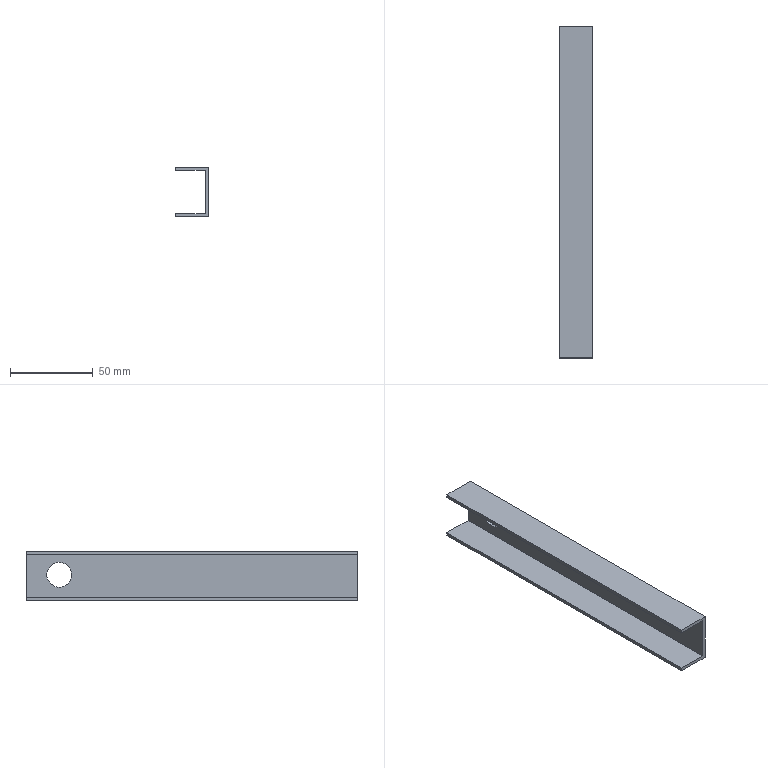Component | SolidWorks | Copy_of_Part4-1 | 1 solid | 12 faces | box 20 x 200 x 30 mm | volume 26047 mm3 | plane 10 | cylinder 2 | commonest cylinder face diameters 15 x2
build123d program:
from build123d import *

# Parameters (mm, degrees)
EXTRUDE_THIN1_DEPTH = 200
SKETCH3_R           = 7.5
CUT_EXTRUDE1_DEPTH  = 254


with BuildPart() as part:
    # Sketch2 → Extrude-Thin1 (new body)
    with BuildSketch(Plane(origin=(0, 0, 0), x_dir=(1, 0, 0), z_dir=(0, 1, 0))):
        Polygon((-173.819, 20), (-173.819, 0), (-143.819, 0), (-143.819, 20), (-145.819, 20), (-145.819, 2), (-171.819, 2), (-171.819, 20), align=None)
    extrude(amount=EXTRUDE_THIN1_DEPTH)

    # Sketch3 → Cut-Extrude1 (cut)
    with BuildSketch(Plane.XY):
        with Locations((-159.526, 179.97)):
            Circle(SKETCH3_R)
    extrude(amount=-CUT_EXTRUDE1_DEPTH, mode=Mode.SUBTRACT)


solid = part.part

# Placed as in the assembly
solid = solid.moved(Location((152, 30, 167.715), (0, 90, 0)))
STEP:
#1=CARTESIAN_POINT('',(5.906,8.267,13.179));
#2=VERTEX_POINT('',#1);
#3=CARTESIAN_POINT('',(5.906,8.267,12.588));
#4=VERTEX_POINT('',#3);
#5=CARTESIAN_POINT('',(5.906,8.267,12.884));
#6=DIRECTION('',(1.,0.,0.));
#7=DIRECTION('',(0.,0.,-1.));
#8=AXIS2_PLACEMENT_3D('',#5,#6,#7);
#9=CIRCLE('',#8,0.2953);
#10=EDGE_CURVE('',#2,#4,#9,.T.);
#11=ORIENTED_EDGE('',*,*,#10,.F.);
#12=CARTESIAN_POINT('',(5.984,8.267,13.179));
#13=VERTEX_POINT('',#12);
#14=CARTESIAN_POINT('',(-4.016,8.267,13.179));
#15=DIRECTION('',(1.,0.,0.));
#16=VECTOR('',#15,39.37);
#17=LINE('',#14,#16);
#18=EDGE_CURVE('',#2,#13,#17,.T.);
#19=ORIENTED_EDGE('',*,*,#18,.T.);
#20=CARTESIAN_POINT('',(5.984,8.267,12.588));
#21=VERTEX_POINT('',#20);
#22=CARTESIAN_POINT('',(5.984,8.267,12.884));
#23=DIRECTION('',(1.,0.,0.));
#24=DIRECTION('',(0.,0.,-1.));
#25=AXIS2_PLACEMENT_3D('',#22,#23,#24);
#26=CIRCLE('',#25,0.2953);
#27=EDGE_CURVE('',#13,#21,#26,.T.);
#28=ORIENTED_EDGE('',*,*,#27,.T.);
#29=CARTESIAN_POINT('',(-4.016,8.267,12.588));
#30=DIRECTION('',(1.,0.,0.));
#31=VECTOR('',#30,39.37);
#32=LINE('',#29,#31);
#33=EDGE_CURVE('',#4,#21,#32,.T.);
#34=ORIENTED_EDGE('',*,*,#33,.F.);
#35=EDGE_LOOP('',(#11,#19,#28,#34));
#36=FACE_OUTER_BOUND('',#35,.T.);
#37=CARTESIAN_POINT('',(-4.016,8.267,12.884));
#38=DIRECTION('',(1.,0.,0.));
#39=DIRECTION('',(0.,0.,-1.));
#40=AXIS2_PLACEMENT_3D('',#37,#38,#39);
#41=CYLINDRICAL_SURFACE('',#40,0.2953);
#42=ADVANCED_FACE('',(#36),#41,.F.);
#43=CARTESIAN_POINT('',(5.906,1.181,13.367));
#44=VERTEX_POINT('',#43);
#45=CARTESIAN_POINT('',(5.197,1.181,13.367));
#46=VERTEX_POINT('',#45);
#47=CARTESIAN_POINT('',(5.197,1.181,13.367));
#48=DIRECTION('',(-1.,0.,0.));
#49=VECTOR('',#48,39.37);
#50=LINE('',#47,#49);
#51=EDGE_CURVE('',#44,#46,#50,.T.);
#52=ORIENTED_EDGE('',*,*,#51,.T.);
#53=CARTESIAN_POINT('',(5.197,9.055,13.367));
#54=VERTEX_POINT('',#53);
#55=CARTESIAN_POINT('',(5.197,9.055,13.367));
#56=DIRECTION('',(0.,-1.,0.));
#57=VECTOR('',#56,39.37);
#58=LINE('',#55,#57);
#59=EDGE_CURVE('',#54,#46,#58,.T.);
#60=ORIENTED_EDGE('',*,*,#59,.F.);
#61=CARTESIAN_POINT('',(5.906,9.055,13.367));
#62=VERTEX_POINT('',#61);
#63=CARTESIAN_POINT('',(5.197,9.055,13.367));
#64=DIRECTION('',(-1.,0.,0.));
#65=VECTOR('',#64,39.37);
#66=LINE('',#63,#65);
#67=EDGE_CURVE('',#62,#54,#66,.T.);
#68=ORIENTED_EDGE('',*,*,#67,.F.);
#69=CARTESIAN_POINT('',(5.906,9.055,13.367));
#70=DIRECTION('',(0.,-1.,0.));
#71=VECTOR('',#70,39.37);
#72=LINE('',#69,#71);
#73=EDGE_CURVE('',#62,#44,#72,.T.);
#74=ORIENTED_EDGE('',*,*,#73,.T.);
#75=EDGE_LOOP('',(#52,#60,#68,#74));
#76=FACE_OUTER_BOUND('',#75,.T.);
#77=CARTESIAN_POINT('',(5.197,9.055,13.367));
#78=DIRECTION('',(0.,0.,1.));
#79=DIRECTION('',(1.,0.,0.));
#80=AXIS2_PLACEMENT_3D('',#77,#78,#79);
#81=PLANE('',#80);
#82=ADVANCED_FACE('',(#76),#81,.F.);
#83=CARTESIAN_POINT('',(5.197,1.181,13.446));
#84=VERTEX_POINT('',#83);
#85=CARTESIAN_POINT('',(5.197,1.181,13.446));
#86=DIRECTION('',(0.,0.,-1.));
#87=VECTOR('',#86,39.37);
#88=LINE('',#85,#87);
#89=EDGE_CURVE('',#84,#46,#88,.T.);
#90=ORIENTED_EDGE('',*,*,#89,.F.);
#91=CARTESIAN_POINT('',(5.197,9.055,13.446));
#92=VERTEX_POINT('',#91);
#93=CARTESIAN_POINT('',(5.197,9.055,13.446));
#94=DIRECTION('',(0.,-1.,0.));
#95=VECTOR('',#94,39.37);
#96=LINE('',#93,#95);
#97=EDGE_CURVE('',#92,#84,#96,.T.);
#98=ORIENTED_EDGE('',*,*,#97,.F.);
#99=CARTESIAN_POINT('',(5.197,9.055,13.446));
#100=DIRECTION('',(0.,0.,-1.));
#101=VECTOR('',#100,39.37);
#102=LINE('',#99,#101);
#103=EDGE_CURVE('',#92,#54,#102,.T.);
#104=ORIENTED_EDGE('',*,*,#103,.T.);
#105=ORIENTED_EDGE('',*,*,#59,.T.);
#106=EDGE_LOOP('',(#90,#98,#104,#105));
#107=FACE_OUTER_BOUND('',#106,.T.);
#108=CARTESIAN_POINT('',(5.197,9.055,13.446));
#109=DIRECTION('',(-1.,0.,0.));
#110=DIRECTION('',(0.,0.,1.));
#111=AXIS2_PLACEMENT_3D('',#108,#109,#110);
#112=PLANE('',#111);
#113=ADVANCED_FACE('',(#107),#112,.T.);
#114=CARTESIAN_POINT('',(5.984,1.181,13.446));
#115=VERTEX_POINT('',#114);
#116=CARTESIAN_POINT('',(5.197,1.181,13.446));
#117=DIRECTION('',(-1.,0.,0.));
#118=VECTOR('',#117,39.37);
#119=LINE('',#116,#118);
#120=EDGE_CURVE('',#115,#84,#119,.T.);
#121=ORIENTED_EDGE('',*,*,#120,.F.);
#122=CARTESIAN_POINT('',(5.984,9.055,13.446));
#123=VERTEX_POINT('',#122);
#124=CARTESIAN_POINT('',(5.984,9.055,13.446));
#125=DIRECTION('',(0.,-1.,0.));
#126=VECTOR('',#125,39.37);
#127=LINE('',#124,#126);
#128=EDGE_CURVE('',#123,#115,#127,.T.);
#129=ORIENTED_EDGE('',*,*,#128,.F.);
#130=CARTESIAN_POINT('',(5.197,9.055,13.446));
#131=DIRECTION('',(-1.,0.,0.));
#132=VECTOR('',#131,39.37);
#133=LINE('',#130,#132);
#134=EDGE_CURVE('',#123,#92,#133,.T.);
#135=ORIENTED_EDGE('',*,*,#134,.T.);
#136=ORIENTED_EDGE('',*,*,#97,.T.);
#137=EDGE_LOOP('',(#121,#129,#135,#136));
#138=FACE_OUTER_BOUND('',#137,.T.);
#139=CARTESIAN_POINT('',(5.197,9.055,13.446));
#140=DIRECTION('',(0.,0.,1.));
#141=DIRECTION('',(1.,0.,0.));
#142=AXIS2_PLACEMENT_3D('',#139,#140,#141);
#143=PLANE('',#142);
#144=ADVANCED_FACE('',(#138),#143,.T.);
#145=CARTESIAN_POINT('',(5.984,8.267,12.884));
#146=DIRECTION('',(1.,0.,0.));
#147=DIRECTION('',(0.,0.,-1.));
#148=AXIS2_PLACEMENT_3D('',#145,#146,#147);
#149=CIRCLE('',#148,0.2953);
#150=EDGE_CURVE('',#21,#13,#149,.T.);
#151=ORIENTED_EDGE('',*,*,#150,.F.);
#152=ORIENTED_EDGE('',*,*,#27,.F.);
#153=EDGE_LOOP('',(#151,#152));
#154=FACE_BOUND('',#153,.T.);
#155=CARTESIAN_POINT('',(5.984,1.181,12.265));
#156=VERTEX_POINT('',#155);
#157=CARTESIAN_POINT('',(5.984,1.181,13.446));
#158=DIRECTION('',(0.,0.,1.));
#159=VECTOR('',#158,39.37);
#160=LINE('',#157,#159);
#161=EDGE_CURVE('',#156,#115,#160,.T.);
#162=ORIENTED_EDGE('',*,*,#161,.F.);
#163=CARTESIAN_POINT('',(5.984,9.055,12.265));
#164=VERTEX_POINT('',#163);
#165=CARTESIAN_POINT('',(5.984,9.055,12.265));
#166=DIRECTION('',(0.,-1.,0.));
#167=VECTOR('',#166,39.37);
#168=LINE('',#165,#167);
#169=EDGE_CURVE('',#164,#156,#168,.T.);
#170=ORIENTED_EDGE('',*,*,#169,.F.);
#171=CARTESIAN_POINT('',(5.984,9.055,13.446));
#172=DIRECTION('',(0.,0.,1.));
#173=VECTOR('',#172,39.37);
#174=LINE('',#171,#173);
#175=EDGE_CURVE('',#164,#123,#174,.T.);
#176=ORIENTED_EDGE('',*,*,#175,.T.);
#177=ORIENTED_EDGE('',*,*,#128,.T.);
#178=EDGE_LOOP('',(#162,#170,#176,#177));
#179=FACE_OUTER_BOUND('',#178,.T.);
#180=CARTESIAN_POINT('',(5.984,9.055,13.446));
#181=DIRECTION('',(1.,0.,0.));
#182=DIRECTION('',(0.,0.,-1.));
#183=AXIS2_PLACEMENT_3D('',#180,#181,#182);
#184=PLANE('',#183);
#185=ADVANCED_FACE('',(#154,#179),#184,.T.);
#186=CARTESIAN_POINT('',(5.197,1.181,12.265));
#187=VERTEX_POINT('',#186);
#188=CARTESIAN_POINT('',(5.197,1.181,12.265));
#189=DIRECTION('',(1.,0.,0.));
#190=VECTOR('',#189,39.37);
#191=LINE('',#188,#190);
#192=EDGE_CURVE('',#187,#156,#191,.T.);
#193=ORIENTED_EDGE('',*,*,#192,.F.);
#194=CARTESIAN_POINT('',(5.197,9.055,12.265));
#195=VERTEX_POINT('',#194);
#196=CARTESIAN_POINT('',(5.197,9.055,12.265));
#197=DIRECTION('',(0.,-1.,0.));
#198=VECTOR('',#197,39.37);
#199=LINE('',#196,#198);
#200=EDGE_CURVE('',#195,#187,#199,.T.);
#201=ORIENTED_EDGE('',*,*,#200,.F.);
#202=CARTESIAN_POINT('',(5.197,9.055,12.265));
#203=DIRECTION('',(1.,0.,0.));
#204=VECTOR('',#203,39.37);
#205=LINE('',#202,#204);
#206=EDGE_CURVE('',#195,#164,#205,.T.);
#207=ORIENTED_EDGE('',*,*,#206,.T.);
#208=ORIENTED_EDGE('',*,*,#169,.T.);
#209=EDGE_LOOP('',(#193,#201,#207,#208));
#210=FACE_OUTER_BOUND('',#209,.T.);
#211=CARTESIAN_POINT('',(5.197,9.055,12.265));
#212=DIRECTION('',(0.,0.,-1.));
#213=DIRECTION('',(-1.,0.,0.));
#214=AXIS2_PLACEMENT_3D('',#211,#212,#213);
#215=PLANE('',#214);
#216=ADVANCED_FACE('',(#210),#215,.T.);
#217=CARTESIAN_POINT('',(5.197,1.181,12.344));
#218=VERTEX_POINT('',#217);
#219=CARTESIAN_POINT('',(5.197,1.181,12.344));
#220=DIRECTION('',(0.,0.,-1.));
#221=VECTOR('',#220,39.37);
#222=LINE('',#219,#221);
#223=EDGE_CURVE('',#218,#187,#222,.T.);
#224=ORIENTED_EDGE('',*,*,#223,.F.);
#225=CARTESIAN_POINT('',(5.197,9.055,12.344));
#226=VERTEX_POINT('',#225);
#227=CARTESIAN_POINT('',(5.197,9.055,12.344));
#228=DIRECTION('',(0.,-1.,0.));
#229=VECTOR('',#228,39.37);
#230=LINE('',#227,#229);
#231=EDGE_CURVE('',#226,#218,#230,.T.);
#232=ORIENTED_EDGE('',*,*,#231,.F.);
#233=CARTESIAN_POINT('',(5.197,9.055,12.344));
#234=DIRECTION('',(0.,0.,-1.));
#235=VECTOR('',#234,39.37);
#236=LINE('',#233,#235);
#237=EDGE_CURVE('',#226,#195,#236,.T.);
#238=ORIENTED_EDGE('',*,*,#237,.T.);
#239=ORIENTED_EDGE('',*,*,#200,.T.);
#240=EDGE_LOOP('',(#224,#232,#238,#239));
#241=FACE_OUTER_BOUND('',#240,.T.);
#242=CARTESIAN_POINT('',(5.197,9.055,12.344));
#243=DIRECTION('',(-1.,0.,0.));
#244=DIRECTION('',(0.,0.,1.));
#245=AXIS2_PLACEMENT_3D('',#242,#243,#244);
#246=PLANE('',#245);
#247=ADVANCED_FACE('',(#241),#246,.T.);
#248=CARTESIAN_POINT('',(5.906,1.181,12.344));
#249=VERTEX_POINT('',#248);
#250=CARTESIAN_POINT('',(5.197,1.181,12.344));
#251=DIRECTION('',(1.,0.,0.));
#252=VECTOR('',#251,39.37);
#253=LINE('',#250,#252);
#254=EDGE_CURVE('',#218,#249,#253,.T.);
#255=ORIENTED_EDGE('',*,*,#254,.T.);
#256=CARTESIAN_POINT('',(5.906,9.055,12.344));
#257=VERTEX_POINT('',#256);
#258=CARTESIAN_POINT('',(5.906,9.055,12.344));
#259=DIRECTION('',(0.,-1.,0.));
#260=VECTOR('',#259,39.37);
#261=LINE('',#258,#260);
#262=EDGE_CURVE('',#257,#249,#261,.T.);
#263=ORIENTED_EDGE('',*,*,#262,.F.);
#264=CARTESIAN_POINT('',(5.197,9.055,12.344));
#265=DIRECTION('',(1.,0.,0.));
#266=VECTOR('',#265,39.37);
#267=LINE('',#264,#266);
#268=EDGE_CURVE('',#226,#257,#267,.T.);
#269=ORIENTED_EDGE('',*,*,#268,.F.);
#270=ORIENTED_EDGE('',*,*,#231,.T.);
#271=EDGE_LOOP('',(#255,#263,#269,#270));
#272=FACE_OUTER_BOUND('',#271,.T.);
#273=CARTESIAN_POINT('',(5.197,9.055,12.344));
#274=DIRECTION('',(0.,0.,-1.));
#275=DIRECTION('',(-1.,0.,0.));
#276=AXIS2_PLACEMENT_3D('',#273,#274,#275);
#277=PLANE('',#276);
#278=ADVANCED_FACE('',(#272),#277,.F.);
#279=CARTESIAN_POINT('',(5.906,8.267,12.884));
#280=DIRECTION('',(1.,0.,0.));
#281=DIRECTION('',(0.,0.,-1.));
#282=AXIS2_PLACEMENT_3D('',#279,#280,#281);
#283=CIRCLE('',#282,0.2953);
#284=EDGE_CURVE('',#4,#2,#283,.T.);
#285=ORIENTED_EDGE('',*,*,#284,.T.);
#286=ORIENTED_EDGE('',*,*,#10,.T.);
#287=EDGE_LOOP('',(#285,#286));
#288=FACE_BOUND('',#287,.T.);
#289=CARTESIAN_POINT('',(5.906,1.181,13.446));
#290=DIRECTION('',(0.,0.,1.));
#291=VECTOR('',#290,39.37);
#292=LINE('',#289,#291);
#293=EDGE_CURVE('',#249,#44,#292,.T.);
#294=ORIENTED_EDGE('',*,*,#293,.T.);
#295=ORIENTED_EDGE('',*,*,#73,.F.);
#296=CARTESIAN_POINT('',(5.906,9.055,13.446));
#297=DIRECTION('',(0.,0.,1.));
#298=VECTOR('',#297,39.37);
#299=LINE('',#296,#298);
#300=EDGE_CURVE('',#257,#62,#299,.T.);
#301=ORIENTED_EDGE('',*,*,#300,.F.);
#302=ORIENTED_EDGE('',*,*,#262,.T.);
#303=EDGE_LOOP('',(#294,#295,#301,#302));
#304=FACE_OUTER_BOUND('',#303,.T.);
#305=CARTESIAN_POINT('',(5.906,9.055,13.446));
#306=DIRECTION('',(1.,0.,0.));
#307=DIRECTION('',(0.,0.,-1.));
#308=AXIS2_PLACEMENT_3D('',#305,#306,#307);
#309=PLANE('',#308);
#310=ADVANCED_FACE('',(#288,#304),#309,.F.);
#311=ORIENTED_EDGE('',*,*,#67,.T.);
#312=ORIENTED_EDGE('',*,*,#103,.F.);
#313=ORIENTED_EDGE('',*,*,#134,.F.);
#314=ORIENTED_EDGE('',*,*,#175,.F.);
#315=ORIENTED_EDGE('',*,*,#206,.F.);
#316=ORIENTED_EDGE('',*,*,#237,.F.);
#317=ORIENTED_EDGE('',*,*,#268,.T.);
#318=ORIENTED_EDGE('',*,*,#300,.T.);
#319=EDGE_LOOP('',(#311,#312,#313,#314,#315,#316,#317,#318));
#320=FACE_OUTER_BOUND('',#319,.T.);
#321=CARTESIAN_POINT('',(5.984,9.055,6.603));
#322=DIRECTION('',(0.,-1.,0.));
#323=DIRECTION('',(0.,0.,1.));
#324=AXIS2_PLACEMENT_3D('',#321,#322,#323);
#325=PLANE('',#324);
#326=ADVANCED_FACE('',(#320),#325,.F.);
#327=ORIENTED_EDGE('',*,*,#51,.F.);
#328=ORIENTED_EDGE('',*,*,#293,.F.);
#329=ORIENTED_EDGE('',*,*,#254,.F.);
#330=ORIENTED_EDGE('',*,*,#223,.T.);
#331=ORIENTED_EDGE('',*,*,#192,.T.);
#332=ORIENTED_EDGE('',*,*,#161,.T.);
#333=ORIENTED_EDGE('',*,*,#120,.T.);
#334=ORIENTED_EDGE('',*,*,#89,.T.);
#335=EDGE_LOOP('',(#327,#328,#329,#330,#331,#332,#333,#334));
#336=FACE_OUTER_BOUND('',#335,.T.);
#337=CARTESIAN_POINT('',(5.984,1.181,6.603));
#338=DIRECTION('',(0.,-1.,0.));
#339=DIRECTION('',(0.,0.,1.));
#340=AXIS2_PLACEMENT_3D('',#337,#338,#339);
#341=PLANE('',#340);
#342=ADVANCED_FACE('',(#336),#341,.T.);
#343=ORIENTED_EDGE('',*,*,#18,.F.);
#344=ORIENTED_EDGE('',*,*,#284,.F.);
#345=ORIENTED_EDGE('',*,*,#33,.T.);
#346=ORIENTED_EDGE('',*,*,#150,.T.);
#347=EDGE_LOOP('',(#343,#344,#345,#346));
#348=FACE_OUTER_BOUND('',#347,.T.);
#349=CARTESIAN_POINT('',(-4.016,8.267,12.884));
#350=DIRECTION('',(1.,0.,0.));
#351=DIRECTION('',(0.,0.,-1.));
#352=AXIS2_PLACEMENT_3D('',#349,#350,#351);
#353=CYLINDRICAL_SURFACE('',#352,0.2953);
#354=ADVANCED_FACE('',(#348),#353,.F.);
#355=CLOSED_SHELL('',(#42,#82,#113,#144,#185,#216,#247,#278,#310,#326,#342,#354));
#356=MANIFOLD_SOLID_BREP('',#355);
#357=CARTESIAN_POINT('',(0.,0.,0.));
#358=DIRECTION('',(0.,0.,1.));
#359=DIRECTION('',(1.,0.,0.));
#360=AXIS2_PLACEMENT_3D('',#357,#358,#359);
#361=(LENGTH_UNIT()NAMED_UNIT(*)SI_UNIT($,.METRE.));
#362=LENGTH_MEASURE_WITH_UNIT(LENGTH_MEASURE(0.0254),#361);
#363=DIMENSIONAL_EXPONENTS(1.,0.,0.,0.,0.,0.,0.);
#364=(CONVERSION_BASED_UNIT('',#362)LENGTH_UNIT()NAMED_UNIT(#363));
#365=UNCERTAINTY_MEASURE_WITH_UNIT(LENGTH_MEASURE(0.00001),#364,'','');
#366=(NAMED_UNIT(*)PLANE_ANGLE_UNIT()SI_UNIT($,.RADIAN.));
#367=(NAMED_UNIT(*)SI_UNIT($,.STERADIAN.)SOLID_ANGLE_UNIT());
#368=(GEOMETRIC_REPRESENTATION_CONTEXT(3)GLOBAL_UNCERTAINTY_ASSIGNED_CONTEXT((#365))GLOBAL_UNIT_ASSIGNED_CONTEXT((#364,#366,#367))REPRESENTATION_CONTEXT('',''));
#369=ADVANCED_BREP_SHAPE_REPRESENTATION('',(#356,#360),#368);
#370=COLOUR_RGB('',0.7922,0.8196,0.9333);
#371=FILL_AREA_STYLE_COLOUR('',#370);
#372=FILL_AREA_STYLE('',(#371));
#373=SURFACE_STYLE_FILL_AREA(#372);
#374=SURFACE_SIDE_STYLE('',(#373));
#375=SURFACE_STYLE_USAGE(.BOTH.,#374);
#376=PRESENTATION_STYLE_ASSIGNMENT((#375));
#377=STYLED_ITEM('',(#376),#356);
#378=PRESENTATION_LAYER_ASSIGNMENT('','',(#377));
#379=(LENGTH_UNIT()NAMED_UNIT(*)SI_UNIT($,.METRE.));
#380=LENGTH_MEASURE_WITH_UNIT(LENGTH_MEASURE(0.0254),#379);
#381=DIMENSIONAL_EXPONENTS(1.,0.,0.,0.,0.,0.,0.);
#382=(CONVERSION_BASED_UNIT('',#380)LENGTH_UNIT()NAMED_UNIT(#381));
#383=UNCERTAINTY_MEASURE_WITH_UNIT(LENGTH_MEASURE(0.00001),#382,'','');
#384=(NAMED_UNIT(*)PLANE_ANGLE_UNIT()SI_UNIT($,.RADIAN.));
#385=(NAMED_UNIT(*)SI_UNIT($,.STERADIAN.)SOLID_ANGLE_UNIT());
#386=(GEOMETRIC_REPRESENTATION_CONTEXT(3)GLOBAL_UNCERTAINTY_ASSIGNED_CONTEXT((#383))GLOBAL_UNIT_ASSIGNED_CONTEXT((#382,#384,#385))REPRESENTATION_CONTEXT('',''));
#387=MECHANICAL_DESIGN_GEOMETRIC_PRESENTATION_REPRESENTATION('',(#377),#386);